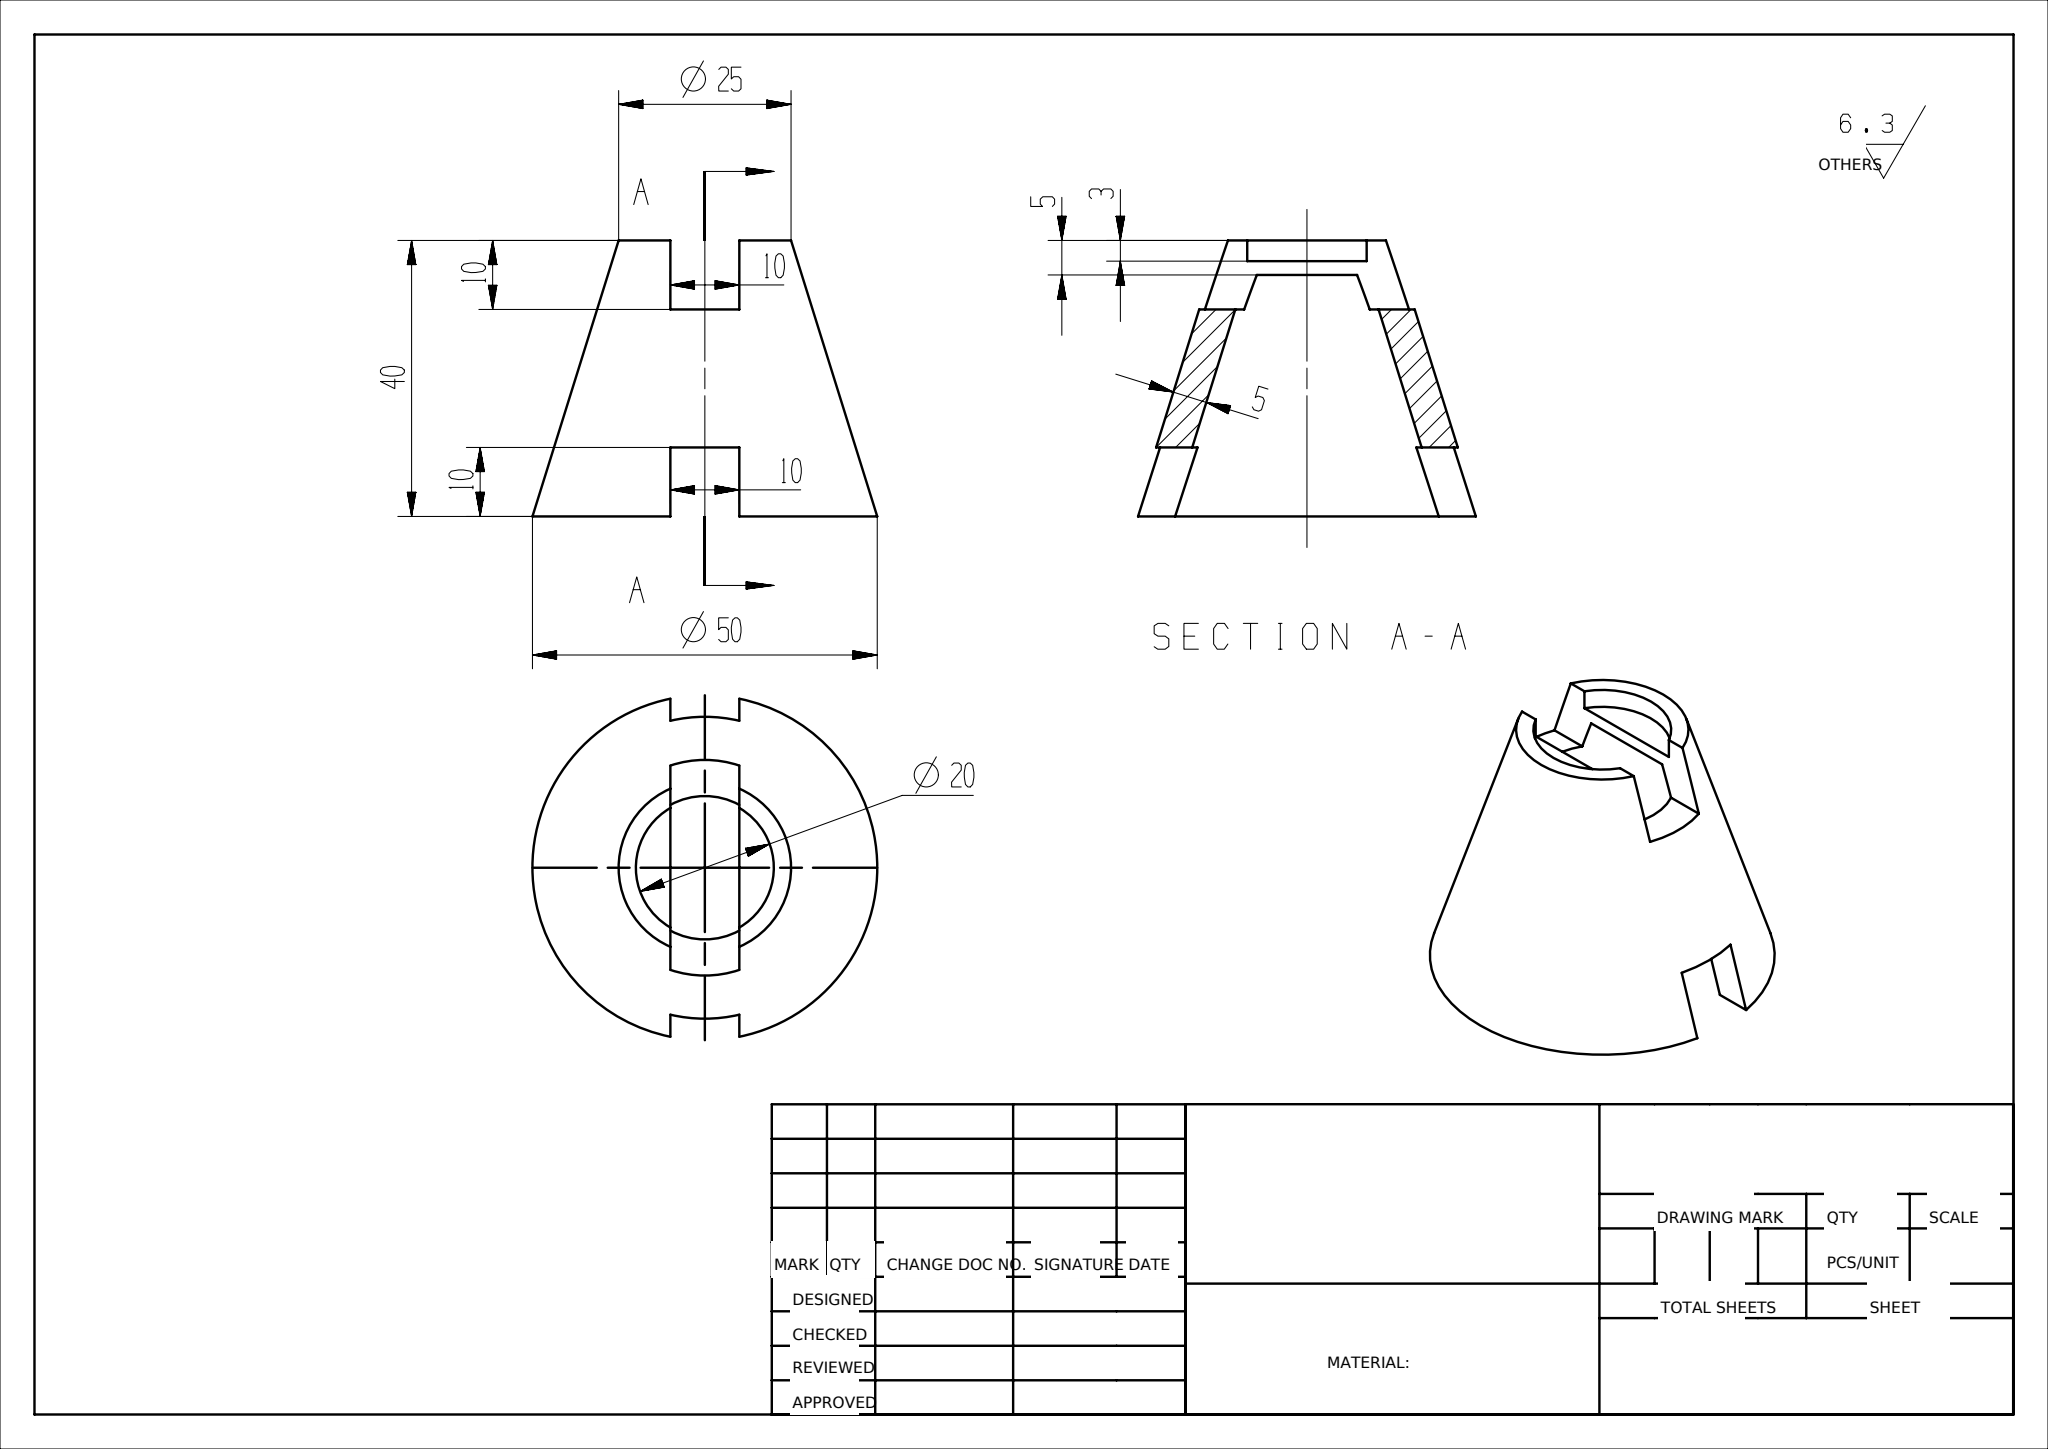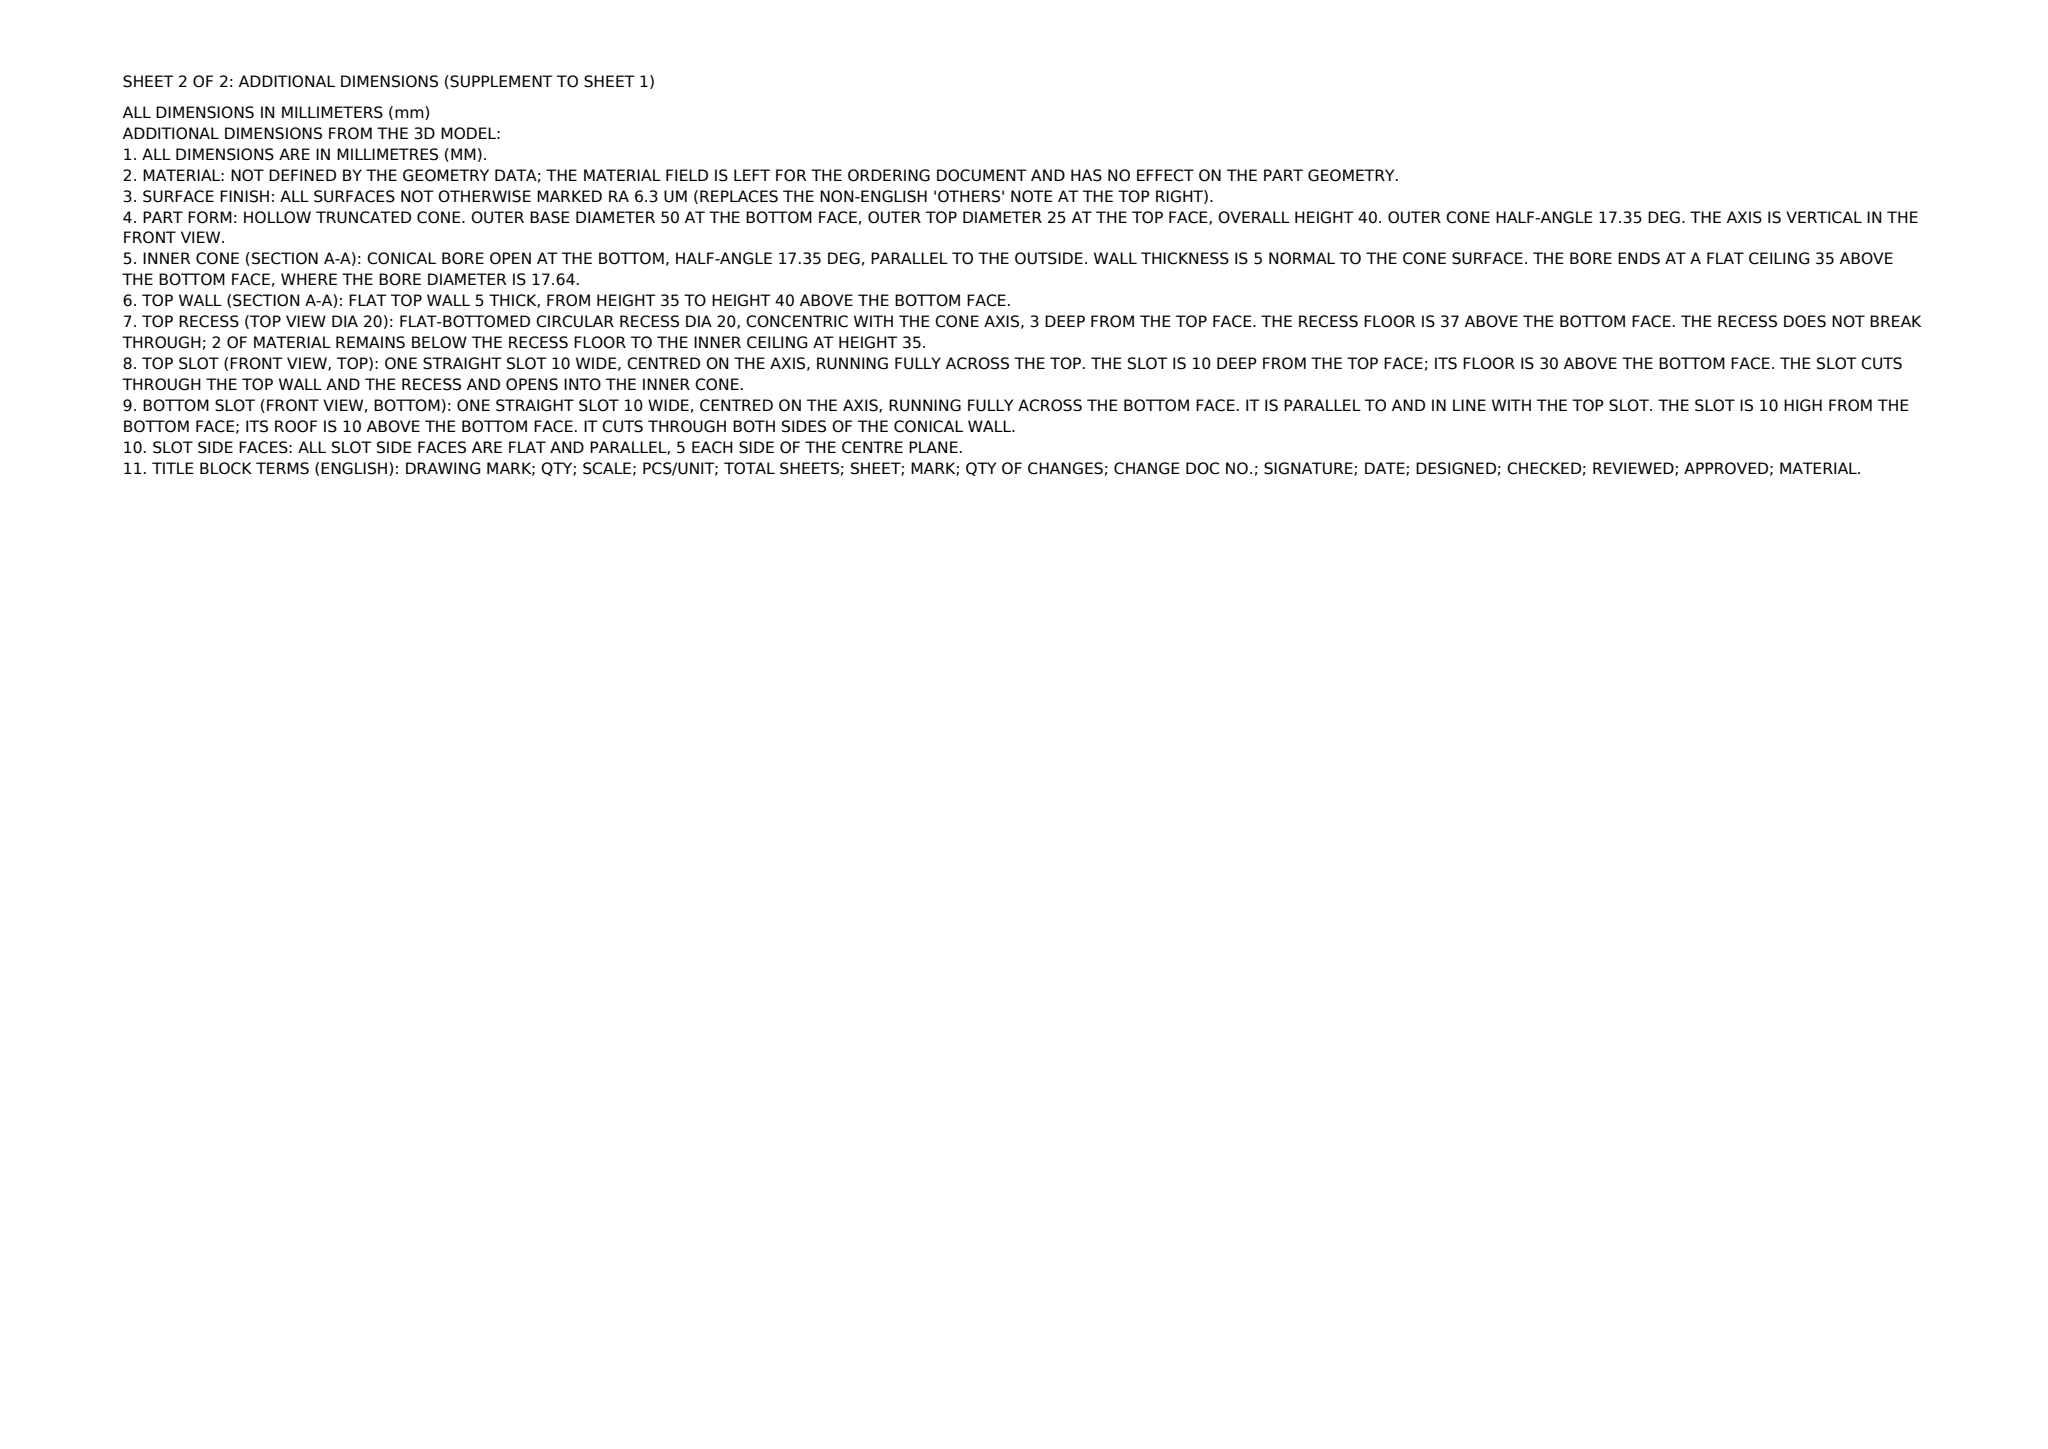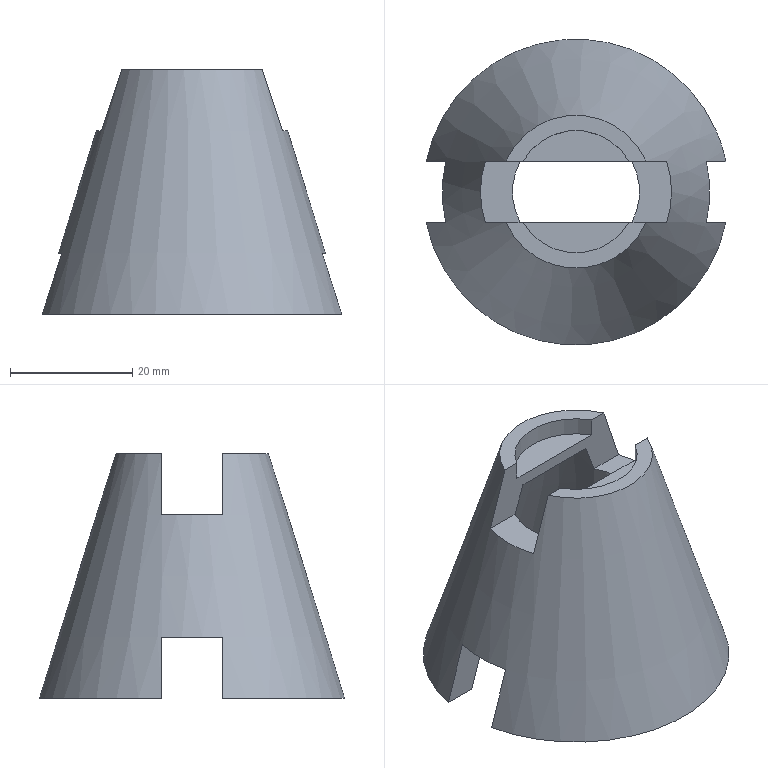Part | NX | mm | 1 solid | 22 faces | box 48.99 x 50 x 40 mm | volume 18996 mm3 | plane 18 | cone 2 | cylinder 2 | commonest cylinder face diameters 20 x2
STEP:
#1=CARTESIAN_POINT('',(0.,0.,0.));
#2=DIRECTION('',(0.,0.,1.));
#3=DIRECTION('',(1.,0.,0.));
#4=AXIS2_PLACEMENT_3D('',#1,#2,#3);
#5=(LENGTH_UNIT()NAMED_UNIT(*)SI_UNIT(.MILLI.,.METRE.));
#6=UNCERTAINTY_MEASURE_WITH_UNIT(LENGTH_MEASURE(0.0508),#5,'','');
#7=(NAMED_UNIT(*)PLANE_ANGLE_UNIT()SI_UNIT($,.RADIAN.));
#8=PLANE_ANGLE_MEASURE_WITH_UNIT(PLANE_ANGLE_MEASURE(0.01745),#7);
#9=DIMENSIONAL_EXPONENTS(0.,0.,0.,0.,0.,0.,0.);
#10=(CONVERSION_BASED_UNIT('',#8)NAMED_UNIT(#9)PLANE_ANGLE_UNIT());
#11=(NAMED_UNIT(*)SI_UNIT($,.STERADIAN.)SOLID_ANGLE_UNIT());
#12=(GEOMETRIC_REPRESENTATION_CONTEXT(3)GLOBAL_UNCERTAINTY_ASSIGNED_CONTEXT((#6))GLOBAL_UNIT_ASSIGNED_CONTEXT((#5,#10,#11))REPRESENTATION_CONTEXT('',''));
#13=SHAPE_REPRESENTATION('',(#4),#12);
#14=CARTESIAN_POINT('',(24.495,-5.,0.));
#15=VERTEX_POINT('',#14);
#16=CARTESIAN_POINT('',(-24.495,-5.,0.));
#17=VERTEX_POINT('',#16);
#18=CARTESIAN_POINT('',(0.,-0.,0.));
#19=DIRECTION('',(0.,-0.,-1.));
#20=DIRECTION('',(0.,1.,-0.));
#21=AXIS2_PLACEMENT_3D('',#18,#19,#20);
#22=CIRCLE('',#21,25.);
#23=EDGE_CURVE('',#15,#17,#22,.T.);
#24=ORIENTED_EDGE('',*,*,#23,.T.);
#25=CARTESIAN_POINT('',(-19.119,-5.,0.));
#26=VERTEX_POINT('',#25);
#27=CARTESIAN_POINT('',(0.,-5.,0.));
#28=DIRECTION('',(1.,0.,0.));
#29=VECTOR('',#28,1.);
#30=LINE('',#27,#29);
#31=EDGE_CURVE('',#17,#26,#30,.T.);
#32=ORIENTED_EDGE('',*,*,#31,.T.);
#33=CARTESIAN_POINT('',(19.119,-5.,0.));
#34=VERTEX_POINT('',#33);
#35=CARTESIAN_POINT('',(0.,-0.,0.));
#36=DIRECTION('',(0.,-0.,-1.));
#37=DIRECTION('',(0.,1.,-0.));
#38=AXIS2_PLACEMENT_3D('',#35,#36,#37);
#39=CIRCLE('',#38,19.762);
#40=EDGE_CURVE('',#34,#26,#39,.T.);
#41=ORIENTED_EDGE('',*,*,#40,.F.);
#42=CARTESIAN_POINT('',(0.,-5.,0.));
#43=DIRECTION('',(1.,0.,0.));
#44=VECTOR('',#43,1.);
#45=LINE('',#42,#44);
#46=EDGE_CURVE('',#34,#15,#45,.T.);
#47=ORIENTED_EDGE('',*,*,#46,.T.);
#48=EDGE_LOOP('',(#24,#32,#41,#47));
#49=FACE_OUTER_BOUND('',#48,.T.);
#50=CARTESIAN_POINT('',(0.,0.,0.));
#51=DIRECTION('',(0.,-0.,-1.));
#52=DIRECTION('',(0.,1.,-0.));
#53=AXIS2_PLACEMENT_3D('',#50,#51,#52);
#54=PLANE('',#53);
#55=ADVANCED_FACE('',(#49),#54,.T.);
#56=CARTESIAN_POINT('',(-24.495,5.,0.));
#57=VERTEX_POINT('',#56);
#58=CARTESIAN_POINT('',(24.495,5.,0.));
#59=VERTEX_POINT('',#58);
#60=CARTESIAN_POINT('',(0.,-0.,0.));
#61=DIRECTION('',(0.,-0.,-1.));
#62=DIRECTION('',(0.,1.,-0.));
#63=AXIS2_PLACEMENT_3D('',#60,#61,#62);
#64=CIRCLE('',#63,25.);
#65=EDGE_CURVE('',#57,#59,#64,.T.);
#66=ORIENTED_EDGE('',*,*,#65,.T.);
#67=CARTESIAN_POINT('',(19.119,5.,0.));
#68=VERTEX_POINT('',#67);
#69=CARTESIAN_POINT('',(0.,5.,0.));
#70=DIRECTION('',(-1.,0.,0.));
#71=VECTOR('',#70,1.);
#72=LINE('',#69,#71);
#73=EDGE_CURVE('',#59,#68,#72,.T.);
#74=ORIENTED_EDGE('',*,*,#73,.T.);
#75=CARTESIAN_POINT('',(-19.119,5.,0.));
#76=VERTEX_POINT('',#75);
#77=CARTESIAN_POINT('',(0.,-0.,0.));
#78=DIRECTION('',(0.,-0.,-1.));
#79=DIRECTION('',(0.,1.,-0.));
#80=AXIS2_PLACEMENT_3D('',#77,#78,#79);
#81=CIRCLE('',#80,19.762);
#82=EDGE_CURVE('',#76,#68,#81,.T.);
#83=ORIENTED_EDGE('',*,*,#82,.F.);
#84=CARTESIAN_POINT('',(0.,5.,0.));
#85=DIRECTION('',(-1.,0.,0.));
#86=VECTOR('',#85,1.);
#87=LINE('',#84,#86);
#88=EDGE_CURVE('',#76,#57,#87,.T.);
#89=ORIENTED_EDGE('',*,*,#88,.T.);
#90=EDGE_LOOP('',(#66,#74,#83,#89));
#91=FACE_OUTER_BOUND('',#90,.T.);
#92=CARTESIAN_POINT('',(0.,0.,0.));
#93=DIRECTION('',(0.,-0.,-1.));
#94=DIRECTION('',(0.,1.,-0.));
#95=AXIS2_PLACEMENT_3D('',#92,#93,#94);
#96=PLANE('',#95);
#97=ADVANCED_FACE('',(#91),#96,.T.);
#98=CARTESIAN_POINT('',(11.456,-5.,40.));
#99=VERTEX_POINT('',#98);
#100=CARTESIAN_POINT('',(14.803,-5.,30.));
#101=VERTEX_POINT('',#100);
#102=CARTESIAN_POINT('',(11.456,-5.,40.));
#103=CARTESIAN_POINT('',(12.591,-5.,36.673));
#104=CARTESIAN_POINT('',(13.702,-5.,33.338));
#105=CARTESIAN_POINT('',(14.803,-5.,30.));
#106=B_SPLINE_CURVE_WITH_KNOTS('',3,(#102,#103,#104,#105),.UNSPECIFIED.,.F.,.F.,(4,4),(0.,1.),.UNSPECIFIED.);
#107=EDGE_CURVE('',#99,#101,#106,.T.);
#108=ORIENTED_EDGE('',*,*,#107,.F.);
#109=CARTESIAN_POINT('',(-11.456,-5.,40.));
#110=VERTEX_POINT('',#109);
#111=CARTESIAN_POINT('',(0.,-0.,40.));
#112=DIRECTION('',(0.,-0.,-1.));
#113=DIRECTION('',(0.,1.,-0.));
#114=AXIS2_PLACEMENT_3D('',#111,#112,#113);
#115=CIRCLE('',#114,12.5);
#116=EDGE_CURVE('',#99,#110,#115,.T.);
#117=ORIENTED_EDGE('',*,*,#116,.T.);
#118=CARTESIAN_POINT('',(-14.803,-5.,30.));
#119=VERTEX_POINT('',#118);
#120=CARTESIAN_POINT('',(-14.803,-5.,30.));
#121=CARTESIAN_POINT('',(-13.702,-5.,33.338));
#122=CARTESIAN_POINT('',(-12.591,-5.,36.673));
#123=CARTESIAN_POINT('',(-11.456,-5.,40.));
#124=B_SPLINE_CURVE_WITH_KNOTS('',3,(#120,#121,#122,#123),.UNSPECIFIED.,.F.,.F.,(4,4),(0.,1.),.UNSPECIFIED.);
#125=EDGE_CURVE('',#119,#110,#124,.T.);
#126=ORIENTED_EDGE('',*,*,#125,.F.);
#127=CARTESIAN_POINT('',(-14.803,5.,30.));
#128=VERTEX_POINT('',#127);
#129=CARTESIAN_POINT('',(0.,-0.,30.));
#130=DIRECTION('',(0.,0.,1.));
#131=DIRECTION('',(-1.,0.,0.));
#132=AXIS2_PLACEMENT_3D('',#129,#130,#131);
#133=CIRCLE('',#132,15.625);
#134=EDGE_CURVE('',#128,#119,#133,.T.);
#135=ORIENTED_EDGE('',*,*,#134,.F.);
#136=CARTESIAN_POINT('',(-11.456,5.,40.));
#137=VERTEX_POINT('',#136);
#138=CARTESIAN_POINT('',(-11.456,5.,40.));
#139=CARTESIAN_POINT('',(-12.591,5.,36.673));
#140=CARTESIAN_POINT('',(-13.702,5.,33.338));
#141=CARTESIAN_POINT('',(-14.803,5.,30.));
#142=B_SPLINE_CURVE_WITH_KNOTS('',3,(#138,#139,#140,#141),.UNSPECIFIED.,.F.,.F.,(4,4),(0.,1.),.UNSPECIFIED.);
#143=EDGE_CURVE('',#137,#128,#142,.T.);
#144=ORIENTED_EDGE('',*,*,#143,.F.);
#145=CARTESIAN_POINT('',(11.456,5.,40.));
#146=VERTEX_POINT('',#145);
#147=CARTESIAN_POINT('',(0.,-0.,40.));
#148=DIRECTION('',(0.,-0.,-1.));
#149=DIRECTION('',(0.,1.,-0.));
#150=AXIS2_PLACEMENT_3D('',#147,#148,#149);
#151=CIRCLE('',#150,12.5);
#152=EDGE_CURVE('',#137,#146,#151,.T.);
#153=ORIENTED_EDGE('',*,*,#152,.T.);
#154=CARTESIAN_POINT('',(14.803,5.,30.));
#155=VERTEX_POINT('',#154);
#156=CARTESIAN_POINT('',(14.803,5.,30.));
#157=CARTESIAN_POINT('',(13.702,5.,33.338));
#158=CARTESIAN_POINT('',(12.591,5.,36.673));
#159=CARTESIAN_POINT('',(11.456,5.,40.));
#160=B_SPLINE_CURVE_WITH_KNOTS('',3,(#156,#157,#158,#159),.UNSPECIFIED.,.F.,.F.,(4,4),(0.,1.),.UNSPECIFIED.);
#161=EDGE_CURVE('',#155,#146,#160,.T.);
#162=ORIENTED_EDGE('',*,*,#161,.F.);
#163=CARTESIAN_POINT('',(0.,-0.,30.));
#164=DIRECTION('',(0.,0.,1.));
#165=DIRECTION('',(-1.,0.,0.));
#166=AXIS2_PLACEMENT_3D('',#163,#164,#165);
#167=CIRCLE('',#166,15.625);
#168=EDGE_CURVE('',#101,#155,#167,.T.);
#169=ORIENTED_EDGE('',*,*,#168,.F.);
#170=EDGE_LOOP('',(#108,#117,#126,#135,#144,#153,#162,#169));
#171=FACE_BOUND('',#170,.T.);
#172=CARTESIAN_POINT('',(-21.296,5.,10.));
#173=VERTEX_POINT('',#172);
#174=CARTESIAN_POINT('',(-21.296,-5.,10.));
#175=VERTEX_POINT('',#174);
#176=CARTESIAN_POINT('',(0.,-0.,10.));
#177=DIRECTION('',(0.,0.,1.));
#178=DIRECTION('',(0.,1.,-0.));
#179=AXIS2_PLACEMENT_3D('',#176,#177,#178);
#180=CIRCLE('',#179,21.875);
#181=EDGE_CURVE('',#173,#175,#180,.T.);
#182=ORIENTED_EDGE('',*,*,#181,.T.);
#183=CARTESIAN_POINT('',(-21.296,-5.,10.));
#184=CARTESIAN_POINT('',(-21.701,-5.,8.739));
#185=CARTESIAN_POINT('',(-22.105,-5.,7.477));
#186=CARTESIAN_POINT('',(-22.509,-5.,6.215));
#187=CARTESIAN_POINT('',(-23.172,-5.,4.144));
#188=CARTESIAN_POINT('',(-23.834,-5.,2.072));
#189=CARTESIAN_POINT('',(-24.495,-5.,0.));
#190=B_SPLINE_CURVE_WITH_KNOTS('',3,(#183,#184,#185,#186,#187,#188,#189),.UNSPECIFIED.,.F.,.F.,(4,3,4),(0.,0.3785,1.),.UNSPECIFIED.);
#191=EDGE_CURVE('',#175,#17,#190,.T.);
#192=ORIENTED_EDGE('',*,*,#191,.T.);
#193=ORIENTED_EDGE('',*,*,#23,.F.);
#194=CARTESIAN_POINT('',(21.296,-5.,10.));
#195=VERTEX_POINT('',#194);
#196=CARTESIAN_POINT('',(24.495,-5.,0.));
#197=CARTESIAN_POINT('',(23.431,-5.,3.334));
#198=CARTESIAN_POINT('',(22.366,-5.,6.668));
#199=CARTESIAN_POINT('',(21.296,-5.,10.));
#200=B_SPLINE_CURVE_WITH_KNOTS('',3,(#196,#197,#198,#199),.UNSPECIFIED.,.F.,.F.,(4,4),(0.,1.),.UNSPECIFIED.);
#201=EDGE_CURVE('',#15,#195,#200,.T.);
#202=ORIENTED_EDGE('',*,*,#201,.T.);
#203=CARTESIAN_POINT('',(21.296,5.,10.));
#204=VERTEX_POINT('',#203);
#205=CARTESIAN_POINT('',(0.,-0.,10.));
#206=DIRECTION('',(0.,0.,1.));
#207=DIRECTION('',(0.,1.,-0.));
#208=AXIS2_PLACEMENT_3D('',#205,#206,#207);
#209=CIRCLE('',#208,21.875);
#210=EDGE_CURVE('',#195,#204,#209,.T.);
#211=ORIENTED_EDGE('',*,*,#210,.T.);
#212=CARTESIAN_POINT('',(21.296,5.,10.));
#213=CARTESIAN_POINT('',(21.701,5.,8.739));
#214=CARTESIAN_POINT('',(22.105,5.,7.477));
#215=CARTESIAN_POINT('',(22.509,5.,6.215));
#216=CARTESIAN_POINT('',(23.172,5.,4.144));
#217=CARTESIAN_POINT('',(23.834,5.,2.072));
#218=CARTESIAN_POINT('',(24.495,5.,0.));
#219=B_SPLINE_CURVE_WITH_KNOTS('',3,(#212,#213,#214,#215,#216,#217,#218),.UNSPECIFIED.,.F.,.F.,(4,3,4),(0.,0.3785,1.),.UNSPECIFIED.);
#220=EDGE_CURVE('',#204,#59,#219,.T.);
#221=ORIENTED_EDGE('',*,*,#220,.T.);
#222=ORIENTED_EDGE('',*,*,#65,.F.);
#223=CARTESIAN_POINT('',(-24.495,5.,0.));
#224=CARTESIAN_POINT('',(-23.431,5.,3.334));
#225=CARTESIAN_POINT('',(-22.366,5.,6.668));
#226=CARTESIAN_POINT('',(-21.296,5.,10.));
#227=B_SPLINE_CURVE_WITH_KNOTS('',3,(#223,#224,#225,#226),.UNSPECIFIED.,.F.,.F.,(4,4),(0.,1.),.UNSPECIFIED.);
#228=EDGE_CURVE('',#57,#173,#227,.T.);
#229=ORIENTED_EDGE('',*,*,#228,.T.);
#230=EDGE_LOOP('',(#182,#192,#193,#202,#211,#221,#222,#229));
#231=FACE_BOUND('',#230,.T.);
#232=CARTESIAN_POINT('',(0.,-0.,0.));
#233=DIRECTION('',(0.,-0.,-1.));
#234=DIRECTION('',(0.,1.,-0.));
#235=AXIS2_PLACEMENT_3D('',#232,#233,#234);
#236=CONICAL_SURFACE('',#235,25.,17.354);
#237=ADVANCED_FACE('',(#171,#231),#236,.T.);
#238=CARTESIAN_POINT('',(7.271,-5.,35.));
#239=VERTEX_POINT('',#238);
#240=CARTESIAN_POINT('',(-7.271,-5.,35.));
#241=VERTEX_POINT('',#240);
#242=CARTESIAN_POINT('',(0.,-0.,35.));
#243=DIRECTION('',(0.,-0.,-1.));
#244=DIRECTION('',(0.,-1.,0.));
#245=AXIS2_PLACEMENT_3D('',#242,#243,#244);
#246=CIRCLE('',#245,8.824);
#247=EDGE_CURVE('',#239,#241,#246,.T.);
#248=ORIENTED_EDGE('',*,*,#247,.F.);
#249=CARTESIAN_POINT('',(9.104,-5.,30.));
#250=VERTEX_POINT('',#249);
#251=CARTESIAN_POINT('',(7.271,-5.,35.));
#252=CARTESIAN_POINT('',(7.9,-5.,33.34));
#253=CARTESIAN_POINT('',(8.508,-5.,31.672));
#254=CARTESIAN_POINT('',(9.104,-5.,30.));
#255=B_SPLINE_CURVE_WITH_KNOTS('',3,(#251,#252,#253,#254),.UNSPECIFIED.,.F.,.F.,(4,4),(0.,1.),.UNSPECIFIED.);
#256=EDGE_CURVE('',#239,#250,#255,.T.);
#257=ORIENTED_EDGE('',*,*,#256,.T.);
#258=CARTESIAN_POINT('',(9.104,5.,30.));
#259=VERTEX_POINT('',#258);
#260=CARTESIAN_POINT('',(0.,-0.,30.));
#261=DIRECTION('',(0.,0.,-1.));
#262=DIRECTION('',(-1.,0.,0.));
#263=AXIS2_PLACEMENT_3D('',#260,#261,#262);
#264=CIRCLE('',#263,10.387);
#265=EDGE_CURVE('',#259,#250,#264,.T.);
#266=ORIENTED_EDGE('',*,*,#265,.F.);
#267=CARTESIAN_POINT('',(7.271,5.,35.));
#268=VERTEX_POINT('',#267);
#269=CARTESIAN_POINT('',(9.104,5.,30.));
#270=CARTESIAN_POINT('',(8.508,5.,31.672));
#271=CARTESIAN_POINT('',(7.9,5.,33.341));
#272=CARTESIAN_POINT('',(7.271,5.,35.));
#273=B_SPLINE_CURVE_WITH_KNOTS('',3,(#269,#270,#271,#272),.UNSPECIFIED.,.F.,.F.,(4,4),(0.,1.),.UNSPECIFIED.);
#274=EDGE_CURVE('',#259,#268,#273,.T.);
#275=ORIENTED_EDGE('',*,*,#274,.T.);
#276=CARTESIAN_POINT('',(-7.271,5.,35.));
#277=VERTEX_POINT('',#276);
#278=CARTESIAN_POINT('',(0.,-0.,35.));
#279=DIRECTION('',(0.,-0.,-1.));
#280=DIRECTION('',(0.,-1.,0.));
#281=AXIS2_PLACEMENT_3D('',#278,#279,#280);
#282=CIRCLE('',#281,8.824);
#283=EDGE_CURVE('',#277,#268,#282,.T.);
#284=ORIENTED_EDGE('',*,*,#283,.F.);
#285=CARTESIAN_POINT('',(-9.104,5.,30.));
#286=VERTEX_POINT('',#285);
#287=CARTESIAN_POINT('',(-7.271,5.,35.));
#288=CARTESIAN_POINT('',(-7.9,5.,33.34));
#289=CARTESIAN_POINT('',(-8.508,5.,31.672));
#290=CARTESIAN_POINT('',(-9.104,5.,30.));
#291=B_SPLINE_CURVE_WITH_KNOTS('',3,(#287,#288,#289,#290),.UNSPECIFIED.,.F.,.F.,(4,4),(0.,1.),.UNSPECIFIED.);
#292=EDGE_CURVE('',#277,#286,#291,.T.);
#293=ORIENTED_EDGE('',*,*,#292,.T.);
#294=CARTESIAN_POINT('',(-9.104,-5.,30.));
#295=VERTEX_POINT('',#294);
#296=CARTESIAN_POINT('',(0.,-0.,30.));
#297=DIRECTION('',(0.,0.,-1.));
#298=DIRECTION('',(-1.,0.,0.));
#299=AXIS2_PLACEMENT_3D('',#296,#297,#298);
#300=CIRCLE('',#299,10.387);
#301=EDGE_CURVE('',#295,#286,#300,.T.);
#302=ORIENTED_EDGE('',*,*,#301,.F.);
#303=CARTESIAN_POINT('',(-9.104,-5.,30.));
#304=CARTESIAN_POINT('',(-8.508,-5.,31.672));
#305=CARTESIAN_POINT('',(-7.9,-5.,33.341));
#306=CARTESIAN_POINT('',(-7.271,-5.,35.));
#307=B_SPLINE_CURVE_WITH_KNOTS('',3,(#303,#304,#305,#306),.UNSPECIFIED.,.F.,.F.,(4,4),(0.,1.),.UNSPECIFIED.);
#308=EDGE_CURVE('',#295,#241,#307,.T.);
#309=ORIENTED_EDGE('',*,*,#308,.T.);
#310=EDGE_LOOP('',(#248,#257,#266,#275,#284,#293,#302,#309));
#311=FACE_BOUND('',#310,.T.);
#312=CARTESIAN_POINT('',(-15.867,-5.,10.));
#313=VERTEX_POINT('',#312);
#314=CARTESIAN_POINT('',(-15.867,-5.,10.));
#315=CARTESIAN_POINT('',(-16.326,-5.,8.6));
#316=CARTESIAN_POINT('',(-16.783,-5.,7.199));
#317=CARTESIAN_POINT('',(-17.239,-5.,5.797));
#318=CARTESIAN_POINT('',(-17.868,-5.,3.866));
#319=CARTESIAN_POINT('',(-18.494,-5.,1.933));
#320=CARTESIAN_POINT('',(-19.119,-5.,0.));
#321=B_SPLINE_CURVE_WITH_KNOTS('',3,(#314,#315,#316,#317,#318,#319,#320),.UNSPECIFIED.,.F.,.F.,(4,3,4),(0.,0.4204,1.),.UNSPECIFIED.);
#322=EDGE_CURVE('',#313,#26,#321,.T.);
#323=ORIENTED_EDGE('',*,*,#322,.F.);
#324=CARTESIAN_POINT('',(-15.867,5.,10.));
#325=VERTEX_POINT('',#324);
#326=CARTESIAN_POINT('',(0.,-0.,10.));
#327=DIRECTION('',(0.,0.,1.));
#328=DIRECTION('',(0.,1.,-0.));
#329=AXIS2_PLACEMENT_3D('',#326,#327,#328);
#330=CIRCLE('',#329,16.637);
#331=EDGE_CURVE('',#325,#313,#330,.T.);
#332=ORIENTED_EDGE('',*,*,#331,.F.);
#333=CARTESIAN_POINT('',(-19.119,5.,0.));
#334=CARTESIAN_POINT('',(-18.041,5.,3.335));
#335=CARTESIAN_POINT('',(-16.959,5.,6.669));
#336=CARTESIAN_POINT('',(-15.867,5.,10.));
#337=B_SPLINE_CURVE_WITH_KNOTS('',3,(#333,#334,#335,#336),.UNSPECIFIED.,.F.,.F.,(4,4),(0.,1.),.UNSPECIFIED.);
#338=EDGE_CURVE('',#76,#325,#337,.T.);
#339=ORIENTED_EDGE('',*,*,#338,.F.);
#340=ORIENTED_EDGE('',*,*,#82,.T.);
#341=CARTESIAN_POINT('',(15.867,5.,10.));
#342=VERTEX_POINT('',#341);
#343=CARTESIAN_POINT('',(15.867,5.,10.));
#344=CARTESIAN_POINT('',(16.326,5.,8.6));
#345=CARTESIAN_POINT('',(16.783,5.,7.199));
#346=CARTESIAN_POINT('',(17.239,5.,5.797));
#347=CARTESIAN_POINT('',(17.868,5.,3.866));
#348=CARTESIAN_POINT('',(18.494,5.,1.933));
#349=CARTESIAN_POINT('',(19.119,5.,0.));
#350=B_SPLINE_CURVE_WITH_KNOTS('',3,(#343,#344,#345,#346,#347,#348,#349),.UNSPECIFIED.,.F.,.F.,(4,3,4),(0.,0.4204,1.),.UNSPECIFIED.);
#351=EDGE_CURVE('',#342,#68,#350,.T.);
#352=ORIENTED_EDGE('',*,*,#351,.F.);
#353=CARTESIAN_POINT('',(15.867,-5.,10.));
#354=VERTEX_POINT('',#353);
#355=CARTESIAN_POINT('',(0.,-0.,10.));
#356=DIRECTION('',(0.,0.,1.));
#357=DIRECTION('',(0.,1.,-0.));
#358=AXIS2_PLACEMENT_3D('',#355,#356,#357);
#359=CIRCLE('',#358,16.637);
#360=EDGE_CURVE('',#354,#342,#359,.T.);
#361=ORIENTED_EDGE('',*,*,#360,.F.);
#362=CARTESIAN_POINT('',(19.119,-5.,0.));
#363=CARTESIAN_POINT('',(18.041,-5.,3.335));
#364=CARTESIAN_POINT('',(16.959,-5.,6.669));
#365=CARTESIAN_POINT('',(15.867,-5.,10.));
#366=B_SPLINE_CURVE_WITH_KNOTS('',3,(#362,#363,#364,#365),.UNSPECIFIED.,.F.,.F.,(4,4),(0.,1.),.UNSPECIFIED.);
#367=EDGE_CURVE('',#34,#354,#366,.T.);
#368=ORIENTED_EDGE('',*,*,#367,.F.);
#369=ORIENTED_EDGE('',*,*,#40,.T.);
#370=EDGE_LOOP('',(#323,#332,#339,#340,#352,#361,#368,#369));
#371=FACE_BOUND('',#370,.T.);
#372=CARTESIAN_POINT('',(0.,-0.,-1.491));
#373=DIRECTION('',(0.,-0.,-1.));
#374=DIRECTION('',(0.,1.,-0.));
#375=AXIS2_PLACEMENT_3D('',#372,#373,#374);
#376=CONICAL_SURFACE('',#375,20.228,17.354);
#377=ADVANCED_FACE('',(#311,#371),#376,.F.);
#378=CARTESIAN_POINT('',(-8.66,-5.,40.));
#379=VERTEX_POINT('',#378);
#380=CARTESIAN_POINT('',(8.66,-5.,40.));
#381=VERTEX_POINT('',#380);
#382=CARTESIAN_POINT('',(0.,0.,40.));
#383=DIRECTION('',(0.,0.,1.));
#384=DIRECTION('',(0.,-1.,0.));
#385=AXIS2_PLACEMENT_3D('',#382,#383,#384);
#386=CIRCLE('',#385,10.);
#387=EDGE_CURVE('',#379,#381,#386,.T.);
#388=ORIENTED_EDGE('',*,*,#387,.F.);
#389=CARTESIAN_POINT('',(0.,-5.,40.));
#390=DIRECTION('',(1.,0.,0.));
#391=VECTOR('',#390,1.);
#392=LINE('',#389,#391);
#393=EDGE_CURVE('',#110,#379,#392,.T.);
#394=ORIENTED_EDGE('',*,*,#393,.F.);
#395=ORIENTED_EDGE('',*,*,#116,.F.);
#396=CARTESIAN_POINT('',(0.,-5.,40.));
#397=DIRECTION('',(1.,0.,0.));
#398=VECTOR('',#397,1.);
#399=LINE('',#396,#398);
#400=EDGE_CURVE('',#381,#99,#399,.T.);
#401=ORIENTED_EDGE('',*,*,#400,.F.);
#402=EDGE_LOOP('',(#388,#394,#395,#401));
#403=FACE_OUTER_BOUND('',#402,.T.);
#404=CARTESIAN_POINT('',(0.,12.5,40.));
#405=DIRECTION('',(0.,0.,1.));
#406=DIRECTION('',(0.,-1.,0.));
#407=AXIS2_PLACEMENT_3D('',#404,#405,#406);
#408=PLANE('',#407);
#409=ADVANCED_FACE('',(#403),#408,.T.);
#410=ORIENTED_EDGE('',*,*,#247,.T.);
#411=CARTESIAN_POINT('',(0.,-5.,35.));
#412=DIRECTION('',(1.,0.,0.));
#413=VECTOR('',#412,1.);
#414=LINE('',#411,#413);
#415=EDGE_CURVE('',#241,#239,#414,.T.);
#416=ORIENTED_EDGE('',*,*,#415,.T.);
#417=EDGE_LOOP('',(#410,#416));
#418=FACE_OUTER_BOUND('',#417,.T.);
#419=CARTESIAN_POINT('',(0.,12.5,35.));
#420=DIRECTION('',(0.,0.,1.));
#421=DIRECTION('',(0.,-1.,0.));
#422=AXIS2_PLACEMENT_3D('',#419,#420,#421);
#423=PLANE('',#422);
#424=ADVANCED_FACE('',(#418),#423,.F.);
#425=CARTESIAN_POINT('',(8.66,5.,40.));
#426=VERTEX_POINT('',#425);
#427=CARTESIAN_POINT('',(-8.66,5.,40.));
#428=VERTEX_POINT('',#427);
#429=CARTESIAN_POINT('',(0.,0.,40.));
#430=DIRECTION('',(0.,0.,1.));
#431=DIRECTION('',(0.,-1.,0.));
#432=AXIS2_PLACEMENT_3D('',#429,#430,#431);
#433=CIRCLE('',#432,10.);
#434=EDGE_CURVE('',#426,#428,#433,.T.);
#435=ORIENTED_EDGE('',*,*,#434,.F.);
#436=CARTESIAN_POINT('',(0.,5.,40.));
#437=DIRECTION('',(-1.,0.,0.));
#438=VECTOR('',#437,1.);
#439=LINE('',#436,#438);
#440=EDGE_CURVE('',#146,#426,#439,.T.);
#441=ORIENTED_EDGE('',*,*,#440,.F.);
#442=ORIENTED_EDGE('',*,*,#152,.F.);
#443=CARTESIAN_POINT('',(0.,5.,40.));
#444=DIRECTION('',(-1.,0.,0.));
#445=VECTOR('',#444,1.);
#446=LINE('',#443,#445);
#447=EDGE_CURVE('',#428,#137,#446,.T.);
#448=ORIENTED_EDGE('',*,*,#447,.F.);
#449=EDGE_LOOP('',(#435,#441,#442,#448));
#450=FACE_OUTER_BOUND('',#449,.T.);
#451=CARTESIAN_POINT('',(0.,12.5,40.));
#452=DIRECTION('',(0.,0.,1.));
#453=DIRECTION('',(0.,-1.,0.));
#454=AXIS2_PLACEMENT_3D('',#451,#452,#453);
#455=PLANE('',#454);
#456=ADVANCED_FACE('',(#450),#455,.T.);
#457=ORIENTED_EDGE('',*,*,#283,.T.);
#458=CARTESIAN_POINT('',(0.,5.,35.));
#459=DIRECTION('',(1.,0.,0.));
#460=VECTOR('',#459,1.);
#461=LINE('',#458,#460);
#462=EDGE_CURVE('',#277,#268,#461,.T.);
#463=ORIENTED_EDGE('',*,*,#462,.F.);
#464=EDGE_LOOP('',(#457,#463));
#465=FACE_OUTER_BOUND('',#464,.T.);
#466=CARTESIAN_POINT('',(0.,12.5,35.));
#467=DIRECTION('',(0.,0.,1.));
#468=DIRECTION('',(0.,-1.,0.));
#469=AXIS2_PLACEMENT_3D('',#466,#467,#468);
#470=PLANE('',#469);
#471=ADVANCED_FACE('',(#465),#470,.F.);
#472=ORIENTED_EDGE('',*,*,#168,.T.);
#473=CARTESIAN_POINT('',(-45.,5.,30.));
#474=DIRECTION('',(-1.,0.,0.));
#475=VECTOR('',#474,1.);
#476=LINE('',#473,#475);
#477=EDGE_CURVE('',#155,#259,#476,.T.);
#478=ORIENTED_EDGE('',*,*,#477,.T.);
#479=ORIENTED_EDGE('',*,*,#265,.T.);
#480=CARTESIAN_POINT('',(-45.,-5.,30.));
#481=DIRECTION('',(-1.,0.,0.));
#482=VECTOR('',#481,1.);
#483=LINE('',#480,#482);
#484=EDGE_CURVE('',#101,#250,#483,.T.);
#485=ORIENTED_EDGE('',*,*,#484,.F.);
#486=EDGE_LOOP('',(#472,#478,#479,#485));
#487=FACE_OUTER_BOUND('',#486,.T.);
#488=CARTESIAN_POINT('',(-45.,-5.,30.));
#489=DIRECTION('',(0.,0.,-1.));
#490=DIRECTION('',(-1.,0.,0.));
#491=AXIS2_PLACEMENT_3D('',#488,#489,#490);
#492=PLANE('',#491);
#493=ADVANCED_FACE('',(#487),#492,.F.);
#494=ORIENTED_EDGE('',*,*,#134,.T.);
#495=CARTESIAN_POINT('',(-45.,-5.,30.));
#496=DIRECTION('',(-1.,0.,0.));
#497=VECTOR('',#496,1.);
#498=LINE('',#495,#497);
#499=EDGE_CURVE('',#295,#119,#498,.T.);
#500=ORIENTED_EDGE('',*,*,#499,.F.);
#501=ORIENTED_EDGE('',*,*,#301,.T.);
#502=CARTESIAN_POINT('',(-45.,5.,30.));
#503=DIRECTION('',(-1.,0.,0.));
#504=VECTOR('',#503,1.);
#505=LINE('',#502,#504);
#506=EDGE_CURVE('',#286,#128,#505,.T.);
#507=ORIENTED_EDGE('',*,*,#506,.T.);
#508=EDGE_LOOP('',(#494,#500,#501,#507));
#509=FACE_OUTER_BOUND('',#508,.T.);
#510=CARTESIAN_POINT('',(-45.,-5.,30.));
#511=DIRECTION('',(0.,0.,-1.));
#512=DIRECTION('',(-1.,0.,0.));
#513=AXIS2_PLACEMENT_3D('',#510,#511,#512);
#514=PLANE('',#513);
#515=ADVANCED_FACE('',(#509),#514,.F.);
#516=CARTESIAN_POINT('',(8.66,-5.,37.));
#517=VERTEX_POINT('',#516);
#518=CARTESIAN_POINT('',(-8.66,-5.,37.));
#519=VERTEX_POINT('',#518);
#520=CARTESIAN_POINT('',(-45.,-5.,37.));
#521=DIRECTION('',(-1.,0.,0.));
#522=VECTOR('',#521,1.);
#523=LINE('',#520,#522);
#524=EDGE_CURVE('',#517,#519,#523,.T.);
#525=ORIENTED_EDGE('',*,*,#524,.F.);
#526=CARTESIAN_POINT('',(8.66,-5.,37.));
#527=DIRECTION('',(0.,0.,1.));
#528=VECTOR('',#527,1.);
#529=LINE('',#526,#528);
#530=EDGE_CURVE('',#517,#381,#529,.T.);
#531=ORIENTED_EDGE('',*,*,#530,.T.);
#532=ORIENTED_EDGE('',*,*,#400,.T.);
#533=ORIENTED_EDGE('',*,*,#107,.T.);
#534=ORIENTED_EDGE('',*,*,#484,.T.);
#535=ORIENTED_EDGE('',*,*,#256,.F.);
#536=ORIENTED_EDGE('',*,*,#415,.F.);
#537=ORIENTED_EDGE('',*,*,#308,.F.);
#538=ORIENTED_EDGE('',*,*,#499,.T.);
#539=ORIENTED_EDGE('',*,*,#125,.T.);
#540=ORIENTED_EDGE('',*,*,#393,.T.);
#541=CARTESIAN_POINT('',(-8.66,-5.,37.));
#542=DIRECTION('',(0.,0.,-1.));
#543=VECTOR('',#542,1.);
#544=LINE('',#541,#543);
#545=EDGE_CURVE('',#379,#519,#544,.T.);
#546=ORIENTED_EDGE('',*,*,#545,.T.);
#547=EDGE_LOOP('',(#525,#531,#532,#533,#534,#535,#536,#537,#538,#539,#540,#546));
#548=FACE_OUTER_BOUND('',#547,.T.);
#549=CARTESIAN_POINT('',(-45.,-5.,48.421));
#550=DIRECTION('',(0.,-1.,0.));
#551=DIRECTION('',(0.,-0.,-1.));
#552=AXIS2_PLACEMENT_3D('',#549,#550,#551);
#553=PLANE('',#552);
#554=ADVANCED_FACE('',(#548),#553,.F.);
#555=CARTESIAN_POINT('',(-8.66,5.,37.));
#556=VERTEX_POINT('',#555);
#557=CARTESIAN_POINT('',(8.66,5.,37.));
#558=VERTEX_POINT('',#557);
#559=CARTESIAN_POINT('',(-45.,5.,37.));
#560=DIRECTION('',(1.,0.,0.));
#561=VECTOR('',#560,1.);
#562=LINE('',#559,#561);
#563=EDGE_CURVE('',#556,#558,#562,.T.);
#564=ORIENTED_EDGE('',*,*,#563,.F.);
#565=CARTESIAN_POINT('',(-8.66,5.,37.));
#566=DIRECTION('',(0.,0.,1.));
#567=VECTOR('',#566,1.);
#568=LINE('',#565,#567);
#569=EDGE_CURVE('',#556,#428,#568,.T.);
#570=ORIENTED_EDGE('',*,*,#569,.T.);
#571=ORIENTED_EDGE('',*,*,#447,.T.);
#572=ORIENTED_EDGE('',*,*,#143,.T.);
#573=ORIENTED_EDGE('',*,*,#506,.F.);
#574=ORIENTED_EDGE('',*,*,#292,.F.);
#575=ORIENTED_EDGE('',*,*,#462,.T.);
#576=ORIENTED_EDGE('',*,*,#274,.F.);
#577=ORIENTED_EDGE('',*,*,#477,.F.);
#578=ORIENTED_EDGE('',*,*,#161,.T.);
#579=ORIENTED_EDGE('',*,*,#440,.T.);
#580=CARTESIAN_POINT('',(8.66,5.,37.));
#581=DIRECTION('',(0.,0.,-1.));
#582=VECTOR('',#581,1.);
#583=LINE('',#580,#582);
#584=EDGE_CURVE('',#426,#558,#583,.T.);
#585=ORIENTED_EDGE('',*,*,#584,.T.);
#586=EDGE_LOOP('',(#564,#570,#571,#572,#573,#574,#575,#576,#577,#578,#579,#585));
#587=FACE_OUTER_BOUND('',#586,.T.);
#588=CARTESIAN_POINT('',(-45.,5.,30.));
#589=DIRECTION('',(0.,1.,0.));
#590=DIRECTION('',(0.,-0.,1.));
#591=AXIS2_PLACEMENT_3D('',#588,#589,#590);
#592=PLANE('',#591);
#593=ADVANCED_FACE('',(#587),#592,.F.);
#594=CARTESIAN_POINT('',(-45.,5.,10.));
#595=DIRECTION('',(-1.,0.,0.));
#596=VECTOR('',#595,1.);
#597=LINE('',#594,#596);
#598=EDGE_CURVE('',#204,#342,#597,.T.);
#599=ORIENTED_EDGE('',*,*,#598,.T.);
#600=ORIENTED_EDGE('',*,*,#351,.T.);
#601=ORIENTED_EDGE('',*,*,#73,.F.);
#602=ORIENTED_EDGE('',*,*,#220,.F.);
#603=EDGE_LOOP('',(#599,#600,#601,#602));
#604=FACE_OUTER_BOUND('',#603,.T.);
#605=CARTESIAN_POINT('',(-45.,5.,10.));
#606=DIRECTION('',(0.,-1.,0.));
#607=DIRECTION('',(0.,-0.,-1.));
#608=AXIS2_PLACEMENT_3D('',#605,#606,#607);
#609=PLANE('',#608);
#610=ADVANCED_FACE('',(#604),#609,.T.);
#611=CARTESIAN_POINT('',(-45.,-5.,10.));
#612=DIRECTION('',(-1.,0.,0.));
#613=VECTOR('',#612,1.);
#614=LINE('',#611,#613);
#615=EDGE_CURVE('',#195,#354,#614,.T.);
#616=ORIENTED_EDGE('',*,*,#615,.T.);
#617=ORIENTED_EDGE('',*,*,#360,.T.);
#618=ORIENTED_EDGE('',*,*,#598,.F.);
#619=ORIENTED_EDGE('',*,*,#210,.F.);
#620=EDGE_LOOP('',(#616,#617,#618,#619));
#621=FACE_OUTER_BOUND('',#620,.T.);
#622=CARTESIAN_POINT('',(-45.,-5.,10.));
#623=DIRECTION('',(0.,-0.,-1.));
#624=DIRECTION('',(0.,1.,-0.));
#625=AXIS2_PLACEMENT_3D('',#622,#623,#624);
#626=PLANE('',#625);
#627=ADVANCED_FACE('',(#621),#626,.T.);
#628=ORIENTED_EDGE('',*,*,#46,.F.);
#629=ORIENTED_EDGE('',*,*,#367,.T.);
#630=ORIENTED_EDGE('',*,*,#615,.F.);
#631=ORIENTED_EDGE('',*,*,#201,.F.);
#632=EDGE_LOOP('',(#628,#629,#630,#631));
#633=FACE_OUTER_BOUND('',#632,.T.);
#634=CARTESIAN_POINT('',(-45.,-5.,-8.421));
#635=DIRECTION('',(0.,1.,-0.));
#636=DIRECTION('',(0.,0.,1.));
#637=AXIS2_PLACEMENT_3D('',#634,#635,#636);
#638=PLANE('',#637);
#639=ADVANCED_FACE('',(#633),#638,.T.);
#640=CARTESIAN_POINT('',(-45.,-5.,10.));
#641=DIRECTION('',(-1.,0.,0.));
#642=VECTOR('',#641,1.);
#643=LINE('',#640,#642);
#644=EDGE_CURVE('',#313,#175,#643,.T.);
#645=ORIENTED_EDGE('',*,*,#644,.F.);
#646=ORIENTED_EDGE('',*,*,#322,.T.);
#647=ORIENTED_EDGE('',*,*,#31,.F.);
#648=ORIENTED_EDGE('',*,*,#191,.F.);
#649=EDGE_LOOP('',(#645,#646,#647,#648));
#650=FACE_OUTER_BOUND('',#649,.T.);
#651=CARTESIAN_POINT('',(-45.,-5.,-8.421));
#652=DIRECTION('',(0.,1.,-0.));
#653=DIRECTION('',(0.,0.,1.));
#654=AXIS2_PLACEMENT_3D('',#651,#652,#653);
#655=PLANE('',#654);
#656=ADVANCED_FACE('',(#650),#655,.T.);
#657=CARTESIAN_POINT('',(-45.,5.,10.));
#658=DIRECTION('',(-1.,0.,0.));
#659=VECTOR('',#658,1.);
#660=LINE('',#657,#659);
#661=EDGE_CURVE('',#325,#173,#660,.T.);
#662=ORIENTED_EDGE('',*,*,#661,.F.);
#663=ORIENTED_EDGE('',*,*,#331,.T.);
#664=ORIENTED_EDGE('',*,*,#644,.T.);
#665=ORIENTED_EDGE('',*,*,#181,.F.);
#666=EDGE_LOOP('',(#662,#663,#664,#665));
#667=FACE_OUTER_BOUND('',#666,.T.);
#668=CARTESIAN_POINT('',(-45.,-5.,10.));
#669=DIRECTION('',(0.,-0.,-1.));
#670=DIRECTION('',(0.,1.,-0.));
#671=AXIS2_PLACEMENT_3D('',#668,#669,#670);
#672=PLANE('',#671);
#673=ADVANCED_FACE('',(#667),#672,.T.);
#674=ORIENTED_EDGE('',*,*,#88,.F.);
#675=ORIENTED_EDGE('',*,*,#338,.T.);
#676=ORIENTED_EDGE('',*,*,#661,.T.);
#677=ORIENTED_EDGE('',*,*,#228,.F.);
#678=EDGE_LOOP('',(#674,#675,#676,#677));
#679=FACE_OUTER_BOUND('',#678,.T.);
#680=CARTESIAN_POINT('',(-45.,5.,10.));
#681=DIRECTION('',(0.,-1.,0.));
#682=DIRECTION('',(0.,-0.,-1.));
#683=AXIS2_PLACEMENT_3D('',#680,#681,#682);
#684=PLANE('',#683);
#685=ADVANCED_FACE('',(#679),#684,.T.);
#686=ORIENTED_EDGE('',*,*,#563,.T.);
#687=CARTESIAN_POINT('',(0.,0.,37.));
#688=DIRECTION('',(0.,0.,-1.));
#689=DIRECTION('',(1.,0.,0.));
#690=AXIS2_PLACEMENT_3D('',#687,#688,#689);
#691=CIRCLE('',#690,10.);
#692=EDGE_CURVE('',#556,#558,#691,.T.);
#693=ORIENTED_EDGE('',*,*,#692,.F.);
#694=EDGE_LOOP('',(#686,#693));
#695=FACE_OUTER_BOUND('',#694,.T.);
#696=CARTESIAN_POINT('',(0.,0.,37.));
#697=DIRECTION('',(0.,0.,1.));
#698=DIRECTION('',(1.,0.,0.));
#699=AXIS2_PLACEMENT_3D('',#696,#697,#698);
#700=PLANE('',#699);
#701=ADVANCED_FACE('',(#695),#700,.T.);
#702=ORIENTED_EDGE('',*,*,#692,.T.);
#703=ORIENTED_EDGE('',*,*,#584,.F.);
#704=ORIENTED_EDGE('',*,*,#434,.T.);
#705=ORIENTED_EDGE('',*,*,#569,.F.);
#706=EDGE_LOOP('',(#702,#703,#704,#705));
#707=FACE_OUTER_BOUND('',#706,.T.);
#708=CARTESIAN_POINT('',(0.,0.,37.));
#709=DIRECTION('',(0.,0.,1.));
#710=DIRECTION('',(1.,0.,0.));
#711=AXIS2_PLACEMENT_3D('',#708,#709,#710);
#712=CYLINDRICAL_SURFACE('',#711,10.);
#713=ADVANCED_FACE('',(#707),#712,.F.);
#714=CARTESIAN_POINT('',(0.,0.,37.));
#715=DIRECTION('',(0.,0.,-1.));
#716=DIRECTION('',(1.,0.,0.));
#717=AXIS2_PLACEMENT_3D('',#714,#715,#716);
#718=CIRCLE('',#717,10.);
#719=EDGE_CURVE('',#517,#519,#718,.T.);
#720=ORIENTED_EDGE('',*,*,#719,.T.);
#721=ORIENTED_EDGE('',*,*,#545,.F.);
#722=ORIENTED_EDGE('',*,*,#387,.T.);
#723=ORIENTED_EDGE('',*,*,#530,.F.);
#724=EDGE_LOOP('',(#720,#721,#722,#723));
#725=FACE_OUTER_BOUND('',#724,.T.);
#726=CARTESIAN_POINT('',(0.,0.,37.));
#727=DIRECTION('',(0.,0.,1.));
#728=DIRECTION('',(1.,0.,0.));
#729=AXIS2_PLACEMENT_3D('',#726,#727,#728);
#730=CYLINDRICAL_SURFACE('',#729,10.);
#731=ADVANCED_FACE('',(#725),#730,.F.);
#732=ORIENTED_EDGE('',*,*,#524,.T.);
#733=ORIENTED_EDGE('',*,*,#719,.F.);
#734=EDGE_LOOP('',(#732,#733));
#735=FACE_OUTER_BOUND('',#734,.T.);
#736=CARTESIAN_POINT('',(0.,0.,37.));
#737=DIRECTION('',(0.,0.,1.));
#738=DIRECTION('',(1.,0.,0.));
#739=AXIS2_PLACEMENT_3D('',#736,#737,#738);
#740=PLANE('',#739);
#741=ADVANCED_FACE('',(#735),#740,.T.);
#742=CLOSED_SHELL('',(#55,#97,#237,#377,#409,#424,#456,#471,#493,#515,#554,#593,#610,#627,#639,#656,#673,#685,#701,#713,#731,#741));
#743=MANIFOLD_SOLID_BREP('',#742);
#744=ADVANCED_BREP_SHAPE_REPRESENTATION('',(#743),#12);
#745=SHAPE_REPRESENTATION_RELATIONSHIP('','',#13,#744);
#746=PRESENTATION_LAYER_ASSIGNMENT('','',(#743));
#747=COLOUR_RGB('',1.,0.6,0.);
#748=FILL_AREA_STYLE_COLOUR('',#747);
#749=FILL_AREA_STYLE('',(#748));
#750=SURFACE_STYLE_FILL_AREA(#749);
#751=SURFACE_SIDE_STYLE('',(#750));
#752=SURFACE_STYLE_USAGE(.BOTH.,#751);
#753=PRESENTATION_STYLE_ASSIGNMENT((#752));
#754=STYLED_ITEM('',(#753),#743);
#755=MECHANICAL_DESIGN_GEOMETRIC_PRESENTATION_REPRESENTATION('',(#754),#12);